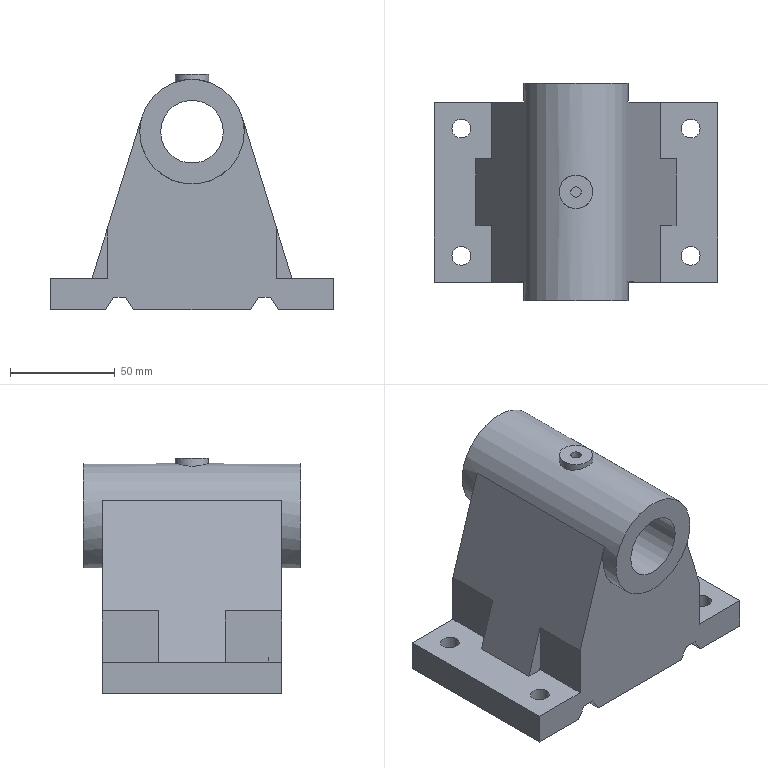Component | NX | TAILSTOCK | 1 solid | 57 faces | volume 417856 mm3 | plane 40 | cylinder 13 | cone 4 | commonest cylinder face diameters 9 x4 3.3 x4 50 x1 30 x1 52 x1 16 x1 5 x1